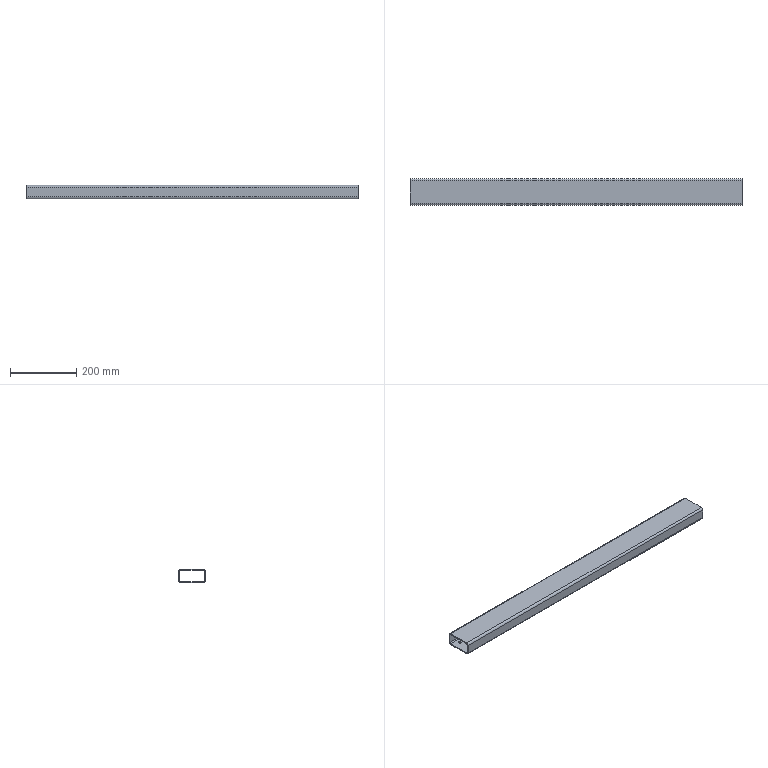Component | SolidWorks | VerticalMovingRectangularTubeWeldment-1_VerticalMovingRectangularTube-4 | 1 solid | 34 faces | volume 659617 mm3 | cylinder 24 | plane 10 | commonest cylinder face diameters 8 x16 12 x4 6 x4 | material Plain Carbon Steel